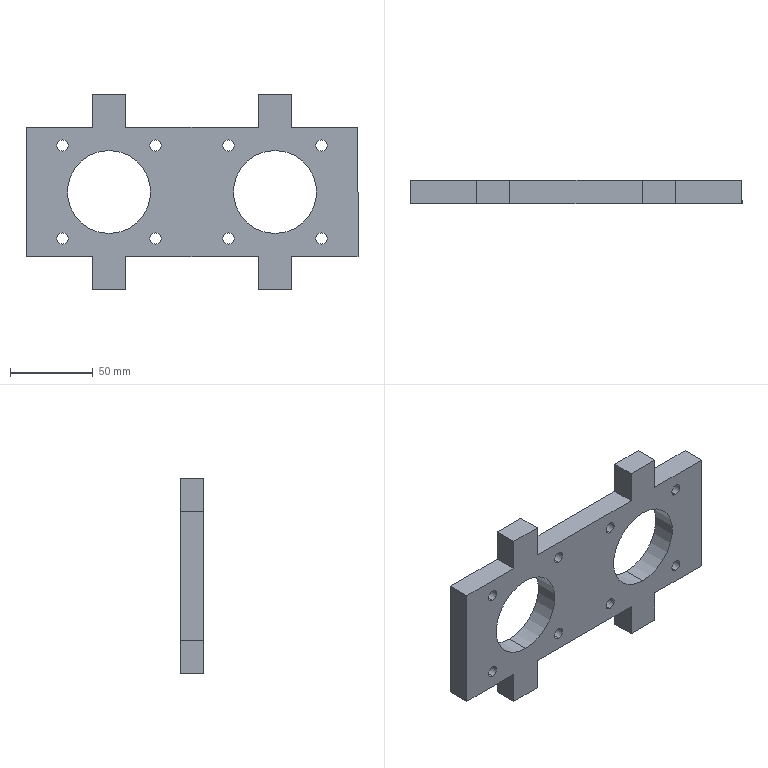Component | SolidWorks | NewTypeCurveBenderReinforcementSeatUpperWheelBox1-DoubleWheel-1 | 1 solid | 82 faces | box 200 x 14 x 118 mm | volume 177572 mm3 | cylinder 36 | plane 30 | cone 16 | commonest cylinder face diameters 6.8 x16 12.5 x16 50 x4
build123d program:
from build123d import *

# Parameters (mm, degrees)
SKETCH1_W                   = 200
SKETCH1_H                   = 78
BOSS_EXTRUDE1_DEPTH         = 14
SKETCH2_R                   = 25
CUT_EXTRUDE1_DEPTH          = 14
SKETCH3_W                   = 20
SKETCH3_H                   = 20
BOSS_EXTRUDE2_DEPTH         = 14
SKETCH7_R                   = 6.25
CUT_EXTRUDE2_DEPTH          = 6
M8_TAPPED_HOLE1_D           = 6.8
M8_TAPPED_HOLE1_CSINK_D     = 8.05
M8_TAPPED_HOLE1_CSINK_ANGLE = 90


with BuildPart() as part:
    # Sketch1 → Boss-Extrude1 (new body)
    with BuildSketch(Plane(origin=(0, 0, 0), x_dir=(1, 0, 0), z_dir=(0, 1, 0))):
        Rectangle(SKETCH1_W, SKETCH1_H)
    extrude(amount=BOSS_EXTRUDE1_DEPTH)

    # Sketch2 → Cut-Extrude1 (cut)
    with BuildSketch(Plane(origin=(0, 14, 0), x_dir=(1, 0, 0), z_dir=(0, 1, 0))):
        with Locations(Location((-50, 0, 0), (0, 0, 270))):
            Circle(SKETCH2_R)
        with Locations(Location((50, 0, 0), (0, 0, 90))):
            Circle(SKETCH2_R)
    extrude(amount=-CUT_EXTRUDE1_DEPTH, mode=Mode.SUBTRACT)

    # Sketch3 → Boss-Extrude2 (add)
    with BuildSketch(Plane(origin=(0, 14, 0), x_dir=(1, 0, 0), z_dir=(0, 1, 0))):
        with Locations((-50, 49)):
            Rectangle(SKETCH3_W, SKETCH3_H)
        with Locations((-50, -49)):
            Rectangle(SKETCH3_W, SKETCH3_H)
        with Locations((50, -49)):
            Rectangle(SKETCH3_W, SKETCH3_H)
        with Locations((50, 49)):
            Rectangle(SKETCH3_W, SKETCH3_H)
    extrude(amount=-BOSS_EXTRUDE2_DEPTH)

    # Sketch7 → Cut-Extrude2 (cut)
    with BuildSketch(Plane.XZ):
        with Locations(Location((-78, -28, 0), (0, 0, 270))):
            Circle(SKETCH7_R)
        with Locations(Location((-78, 28, 0), (0, 0, 270))):
            Circle(SKETCH7_R)
        with Locations(Location((-22, 28, 0), (0, 0, 270))):
            Circle(SKETCH7_R)
        with Locations(Location((22, 28, 0), (0, 0, 270))):
            Circle(SKETCH7_R)
        with Locations(Location((78, 28, 0), (0, 0, 270))):
            Circle(SKETCH7_R)
        with Locations(Location((78, -28, 0), (0, 0, 270))):
            Circle(SKETCH7_R)
        with Locations(Location((22, -28, 0), (0, 0, 270))):
            Circle(SKETCH7_R)
        with Locations(Location((-22, -28, 0), (0, 0, 270))):
            Circle(SKETCH7_R)
    extrude(amount=-CUT_EXTRUDE2_DEPTH, mode=Mode.SUBTRACT)

    # M8 Tapped Hole1 (through all)
    with Locations(Plane(origin=(0, 6, 0), x_dir=(-1, 0, 0), z_dir=(0, -1, 0))):
        with Locations((-78, 28), (-22, 28), (22, 28), (78, 28), (78, -28), (22, -28), (-22, -28), (-78, -28)):
            CounterSinkHole(M8_TAPPED_HOLE1_D / 2, M8_TAPPED_HOLE1_CSINK_D / 2, counter_sink_angle=M8_TAPPED_HOLE1_CSINK_ANGLE)


solid = part.part

# Placed as in the assembly
solid = solid.moved(Location((0, -287, 0), (180, 0, 0)))